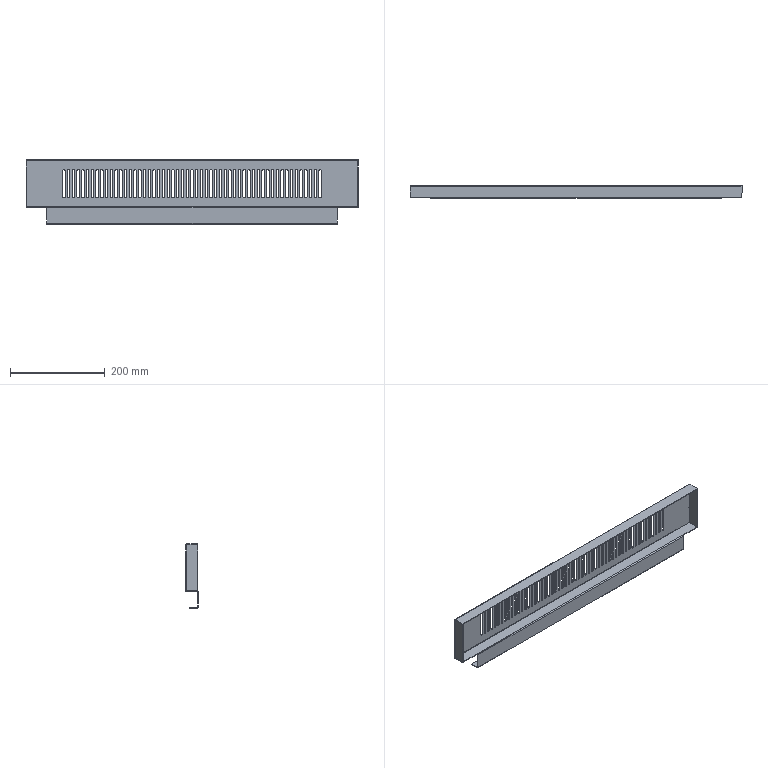Component | SolidWorks | LowerSill-1 | 1 solid | 335 faces | volume 184131 mm3 | cylinder 177 | plane 158 | commonest cylinder face diameters 5 x165 1 x6 4 x6